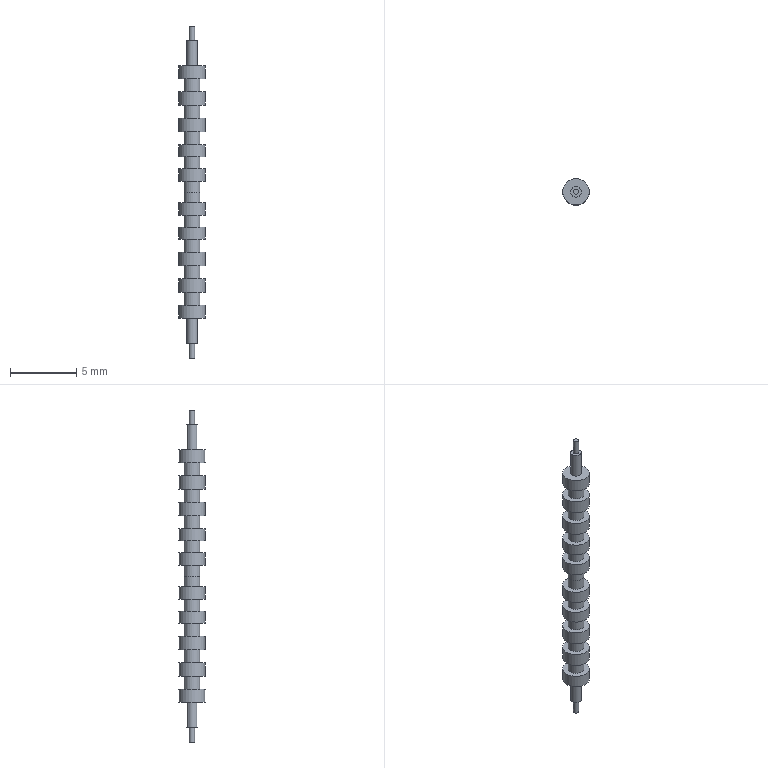Component | NX | MODEL2 | 2 solids | 50 faces | volume 43 mm3 | plane 26 | cylinder 24 | commonest cylinder face diameters 2 x10 1.2 x10 0.8 x2 0.4 x2